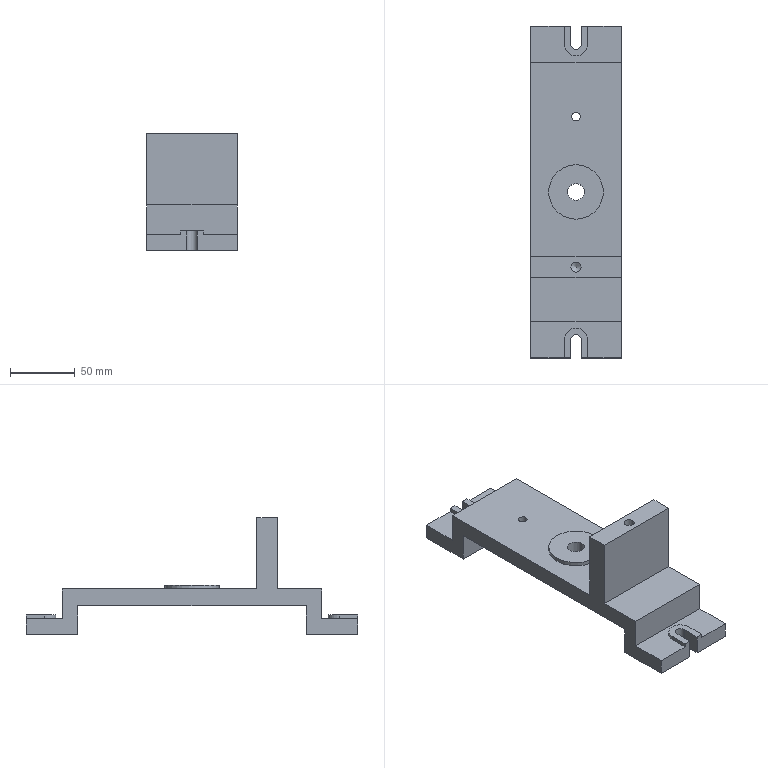Component | NX | FIXTURE_BODY | 1 solid | 42 faces | volume 326142 mm3 | plane 32 | cylinder 9 | cone 1 | commonest cylinder face diameters 8 x2 18 x2 42 x1 13 x1 7.76 x1 6.6 x1 11 x1